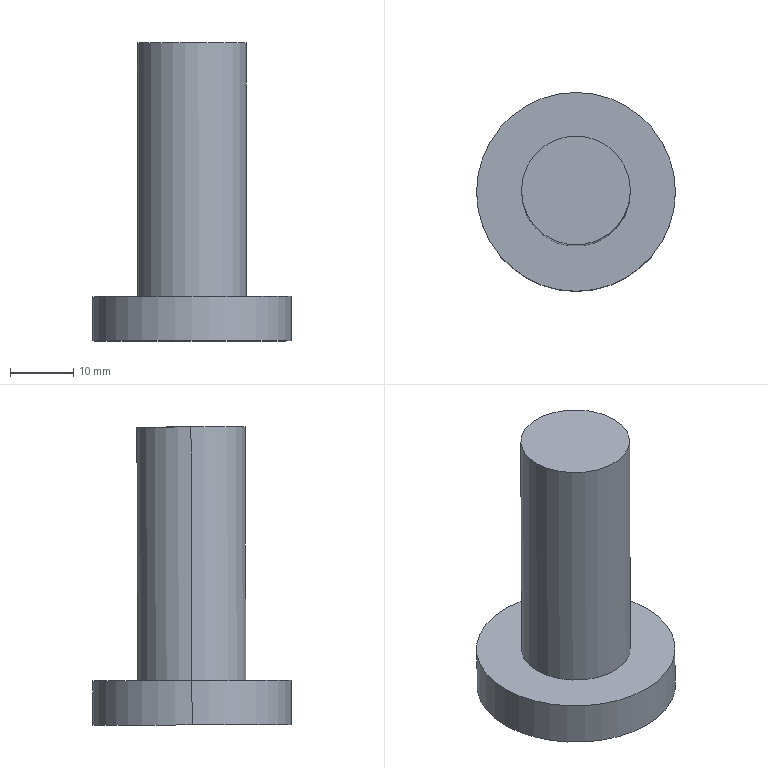Component | SolidWorks | RehabilitationChair-18-11-2 | 1 solid | 7 faces | box 31.35 x 31.37 x 47.09 mm | volume 14682 mm3 | cylinder 4 | plane 3 | commonest cylinder face diameters 17.187 x2 31.344 x2
STEP:
#1=COLOUR_RGB('',0.7922,0.8196,0.9333);
#2=FILL_AREA_STYLE_COLOUR('',#1);
#3=FILL_AREA_STYLE('',(#2));
#4=SURFACE_STYLE_FILL_AREA(#3);
#5=SURFACE_SIDE_STYLE('',(#4));
#6=SURFACE_STYLE_USAGE(.BOTH.,#5);
#7=PRESENTATION_STYLE_ASSIGNMENT((#6));
#8=CARTESIAN_POINT('',(12.381,10.658,14.004));
#9=VERTEX_POINT('',#8);
#10=CARTESIAN_POINT('',(13.057,10.658,14.004));
#11=VERTEX_POINT('',#10);
#12=CARTESIAN_POINT('',(12.719,10.658,14.004));
#13=DIRECTION('',(-0.0003323,0.003798,1.));
#14=DIRECTION('',(-1.,-0.00000716,-0.0003323));
#15=AXIS2_PLACEMENT_3D('',#12,#13,#14);
#16=CIRCLE('',#15,0.3383);
#17=EDGE_CURVE('',#9,#11,#16,.T.);
#18=ORIENTED_EDGE('',*,*,#17,.F.);
#19=CARTESIAN_POINT('',(12.381,10.652,12.429));
#20=VERTEX_POINT('',#19);
#21=CARTESIAN_POINT('',(12.38,10.668,16.801));
#22=DIRECTION('',(0.0003323,-0.003798,-1.));
#23=VECTOR('',#22,39.37);
#24=LINE('',#21,#23);
#25=EDGE_CURVE('',#9,#20,#24,.T.);
#26=ORIENTED_EDGE('',*,*,#25,.T.);
#27=CARTESIAN_POINT('',(13.058,10.652,12.429));
#28=VERTEX_POINT('',#27);
#29=CARTESIAN_POINT('',(12.719,10.652,12.429));
#30=DIRECTION('',(0.0003323,-0.003798,-1.));
#31=DIRECTION('',(1.,0.00000716,0.0003323));
#32=AXIS2_PLACEMENT_3D('',#29,#30,#31);
#33=CIRCLE('',#32,0.3383);
#34=EDGE_CURVE('',#28,#20,#33,.T.);
#35=ORIENTED_EDGE('',*,*,#34,.F.);
#36=CARTESIAN_POINT('',(13.056,10.668,16.801));
#37=DIRECTION('',(0.0003323,-0.003798,-1.));
#38=VECTOR('',#37,39.37);
#39=LINE('',#36,#38);
#40=EDGE_CURVE('',#11,#28,#39,.T.);
#41=ORIENTED_EDGE('',*,*,#40,.F.);
#42=EDGE_LOOP('',(#18,#26,#35,#41));
#43=FACE_OUTER_BOUND('',#42,.T.);
#44=CARTESIAN_POINT('',(12.718,10.668,16.801));
#45=DIRECTION('',(0.0003323,-0.003798,-1.));
#46=DIRECTION('',(1.,0.00000716,0.0003323));
#47=AXIS2_PLACEMENT_3D('',#44,#45,#46);
#48=CYLINDRICAL_SURFACE('',#47,0.3383);
#49=ADVANCED_FACE('',(#43),#48,.T.);
#50=CARTESIAN_POINT('',(13.336,10.651,12.154));
#51=VERTEX_POINT('',#50);
#52=CARTESIAN_POINT('',(12.102,10.651,12.153));
#53=VERTEX_POINT('',#52);
#54=CARTESIAN_POINT('',(12.719,10.651,12.153));
#55=DIRECTION('',(0.0003323,-0.003798,-1.));
#56=DIRECTION('',(1.,0.00000716,0.0003323));
#57=AXIS2_PLACEMENT_3D('',#54,#55,#56);
#58=CIRCLE('',#57,0.617);
#59=EDGE_CURVE('',#51,#53,#58,.T.);
#60=ORIENTED_EDGE('',*,*,#59,.F.);
#61=CARTESIAN_POINT('',(13.336,10.652,12.429));
#62=VERTEX_POINT('',#61);
#63=CARTESIAN_POINT('',(13.336,10.651,12.154));
#64=DIRECTION('',(-0.0003323,0.003798,1.));
#65=VECTOR('',#64,39.37);
#66=LINE('',#63,#65);
#67=EDGE_CURVE('',#51,#62,#66,.T.);
#68=ORIENTED_EDGE('',*,*,#67,.T.);
#69=CARTESIAN_POINT('',(12.102,10.652,12.429));
#70=VERTEX_POINT('',#69);
#71=CARTESIAN_POINT('',(12.719,10.652,12.429));
#72=DIRECTION('',(0.0003323,-0.003798,-1.));
#73=DIRECTION('',(1.,0.00000716,0.0003323));
#74=AXIS2_PLACEMENT_3D('',#71,#72,#73);
#75=CIRCLE('',#74,0.617);
#76=EDGE_CURVE('',#62,#70,#75,.T.);
#77=ORIENTED_EDGE('',*,*,#76,.T.);
#78=CARTESIAN_POINT('',(12.102,10.651,12.153));
#79=DIRECTION('',(-0.0003323,0.003798,1.));
#80=VECTOR('',#79,39.37);
#81=LINE('',#78,#80);
#82=EDGE_CURVE('',#53,#70,#81,.T.);
#83=ORIENTED_EDGE('',*,*,#82,.F.);
#84=EDGE_LOOP('',(#60,#68,#77,#83));
#85=FACE_OUTER_BOUND('',#84,.T.);
#86=CARTESIAN_POINT('',(12.719,10.651,12.153));
#87=DIRECTION('',(-0.0003323,0.003798,1.));
#88=DIRECTION('',(-1.,-0.00000716,-0.0003323));
#89=AXIS2_PLACEMENT_3D('',#86,#87,#88);
#90=CYLINDRICAL_SURFACE('',#89,0.617);
#91=ADVANCED_FACE('',(#85),#90,.T.);
#92=ORIENTED_EDGE('',*,*,#67,.F.);
#93=CARTESIAN_POINT('',(12.719,10.651,12.153));
#94=DIRECTION('',(0.0003323,-0.003798,-1.));
#95=DIRECTION('',(1.,0.00000716,0.0003323));
#96=AXIS2_PLACEMENT_3D('',#93,#94,#95);
#97=CIRCLE('',#96,0.617);
#98=EDGE_CURVE('',#53,#51,#97,.T.);
#99=ORIENTED_EDGE('',*,*,#98,.F.);
#100=ORIENTED_EDGE('',*,*,#82,.T.);
#101=CARTESIAN_POINT('',(12.719,10.652,12.429));
#102=DIRECTION('',(0.0003323,-0.003798,-1.));
#103=DIRECTION('',(1.,0.00000716,0.0003323));
#104=AXIS2_PLACEMENT_3D('',#101,#102,#103);
#105=CIRCLE('',#104,0.617);
#106=EDGE_CURVE('',#70,#62,#105,.T.);
#107=ORIENTED_EDGE('',*,*,#106,.T.);
#108=EDGE_LOOP('',(#92,#99,#100,#107));
#109=FACE_OUTER_BOUND('',#108,.T.);
#110=CARTESIAN_POINT('',(12.719,10.651,12.153));
#111=DIRECTION('',(-0.0003323,0.003798,1.));
#112=DIRECTION('',(-1.,-0.00000716,-0.0003323));
#113=AXIS2_PLACEMENT_3D('',#110,#111,#112);
#114=CYLINDRICAL_SURFACE('',#113,0.617);
#115=ADVANCED_FACE('',(#109),#114,.T.);
#116=ORIENTED_EDGE('',*,*,#98,.T.);
#117=ORIENTED_EDGE('',*,*,#59,.T.);
#118=EDGE_LOOP('',(#116,#117));
#119=FACE_OUTER_BOUND('',#118,.T.);
#120=CARTESIAN_POINT('',(12.719,10.651,12.153));
#121=DIRECTION('',(0.0003323,-0.003798,-1.));
#122=DIRECTION('',(1.,0.00000716,0.0003323));
#123=AXIS2_PLACEMENT_3D('',#120,#121,#122);
#124=PLANE('',#123);
#125=ADVANCED_FACE('',(#119),#124,.T.);
#126=ORIENTED_EDGE('',*,*,#34,.T.);
#127=CARTESIAN_POINT('',(12.719,10.652,12.429));
#128=DIRECTION('',(0.0003323,-0.003798,-1.));
#129=DIRECTION('',(1.,0.00000716,0.0003323));
#130=AXIS2_PLACEMENT_3D('',#127,#128,#129);
#131=CIRCLE('',#130,0.3383);
#132=EDGE_CURVE('',#20,#28,#131,.T.);
#133=ORIENTED_EDGE('',*,*,#132,.T.);
#134=EDGE_LOOP('',(#126,#133));
#135=FACE_BOUND('',#134,.T.);
#136=ORIENTED_EDGE('',*,*,#106,.F.);
#137=ORIENTED_EDGE('',*,*,#76,.F.);
#138=EDGE_LOOP('',(#136,#137));
#139=FACE_OUTER_BOUND('',#138,.T.);
#140=CARTESIAN_POINT('',(12.719,10.652,12.429));
#141=DIRECTION('',(0.0003323,-0.003798,-1.));
#142=DIRECTION('',(1.,0.00000716,0.0003323));
#143=AXIS2_PLACEMENT_3D('',#140,#141,#142);
#144=PLANE('',#143);
#145=ADVANCED_FACE('',(#135,#139),#144,.F.);
#146=CARTESIAN_POINT('',(12.719,10.658,14.004));
#147=DIRECTION('',(-0.0003323,0.003798,1.));
#148=DIRECTION('',(-1.,-0.00000716,-0.0003323));
#149=AXIS2_PLACEMENT_3D('',#146,#147,#148);
#150=CIRCLE('',#149,0.3383);
#151=EDGE_CURVE('',#11,#9,#150,.T.);
#152=ORIENTED_EDGE('',*,*,#151,.T.);
#153=ORIENTED_EDGE('',*,*,#17,.T.);
#154=EDGE_LOOP('',(#152,#153));
#155=FACE_OUTER_BOUND('',#154,.T.);
#156=CARTESIAN_POINT('',(8.099,9.633,14.006));
#157=DIRECTION('',(-0.0003323,0.003798,1.));
#158=DIRECTION('',(-1.,-0.00000716,-0.0003323));
#159=AXIS2_PLACEMENT_3D('',#156,#157,#158);
#160=PLANE('',#159);
#161=ADVANCED_FACE('',(#155),#160,.T.);
#162=ORIENTED_EDGE('',*,*,#25,.F.);
#163=ORIENTED_EDGE('',*,*,#151,.F.);
#164=ORIENTED_EDGE('',*,*,#40,.T.);
#165=ORIENTED_EDGE('',*,*,#132,.F.);
#166=EDGE_LOOP('',(#162,#163,#164,#165));
#167=FACE_OUTER_BOUND('',#166,.T.);
#168=CARTESIAN_POINT('',(12.718,10.668,16.801));
#169=DIRECTION('',(0.0003323,-0.003798,-1.));
#170=DIRECTION('',(1.,0.00000716,0.0003323));
#171=AXIS2_PLACEMENT_3D('',#168,#169,#170);
#172=CYLINDRICAL_SURFACE('',#171,0.3383);
#173=ADVANCED_FACE('',(#167),#172,.T.);
#174=CLOSED_SHELL('',(#49,#91,#115,#125,#145,#161,#173));
#175=MANIFOLD_SOLID_BREP('',#174);
#176=STYLED_ITEM('',(#7),#175);
#177=PRESENTATION_LAYER_ASSIGNMENT('','',(#176));
#178=CARTESIAN_POINT('',(0.,0.,0.));
#179=DIRECTION('',(0.,0.,1.));
#180=DIRECTION('',(1.,0.,0.));
#181=AXIS2_PLACEMENT_3D('',#178,#179,#180);
#182=(LENGTH_UNIT()NAMED_UNIT(*)SI_UNIT($,.METRE.));
#183=LENGTH_MEASURE_WITH_UNIT(LENGTH_MEASURE(0.0254),#182);
#184=DIMENSIONAL_EXPONENTS(1.,0.,0.,0.,0.,0.,0.);
#185=(CONVERSION_BASED_UNIT('',#183)LENGTH_UNIT()NAMED_UNIT(#184));
#186=UNCERTAINTY_MEASURE_WITH_UNIT(LENGTH_MEASURE(0.00001),#185,'','');
#187=(NAMED_UNIT(*)PLANE_ANGLE_UNIT()SI_UNIT($,.RADIAN.));
#188=(NAMED_UNIT(*)SI_UNIT($,.STERADIAN.)SOLID_ANGLE_UNIT());
#189=(GEOMETRIC_REPRESENTATION_CONTEXT(3)GLOBAL_UNCERTAINTY_ASSIGNED_CONTEXT((#186))GLOBAL_UNIT_ASSIGNED_CONTEXT((#185,#187,#188))REPRESENTATION_CONTEXT('',''));
#190=ADVANCED_BREP_SHAPE_REPRESENTATION('',(#175,#181),#189);
#191=(LENGTH_UNIT()NAMED_UNIT(*)SI_UNIT($,.METRE.));
#192=LENGTH_MEASURE_WITH_UNIT(LENGTH_MEASURE(0.0254),#191);
#193=DIMENSIONAL_EXPONENTS(1.,0.,0.,0.,0.,0.,0.);
#194=(CONVERSION_BASED_UNIT('',#192)LENGTH_UNIT()NAMED_UNIT(#193));
#195=UNCERTAINTY_MEASURE_WITH_UNIT(LENGTH_MEASURE(0.00001),#194,'','');
#196=(NAMED_UNIT(*)PLANE_ANGLE_UNIT()SI_UNIT($,.RADIAN.));
#197=(NAMED_UNIT(*)SI_UNIT($,.STERADIAN.)SOLID_ANGLE_UNIT());
#198=(GEOMETRIC_REPRESENTATION_CONTEXT(3)GLOBAL_UNCERTAINTY_ASSIGNED_CONTEXT((#195))GLOBAL_UNIT_ASSIGNED_CONTEXT((#194,#196,#197))REPRESENTATION_CONTEXT('',''));
#199=MECHANICAL_DESIGN_GEOMETRIC_PRESENTATION_REPRESENTATION('',(#176),#198);